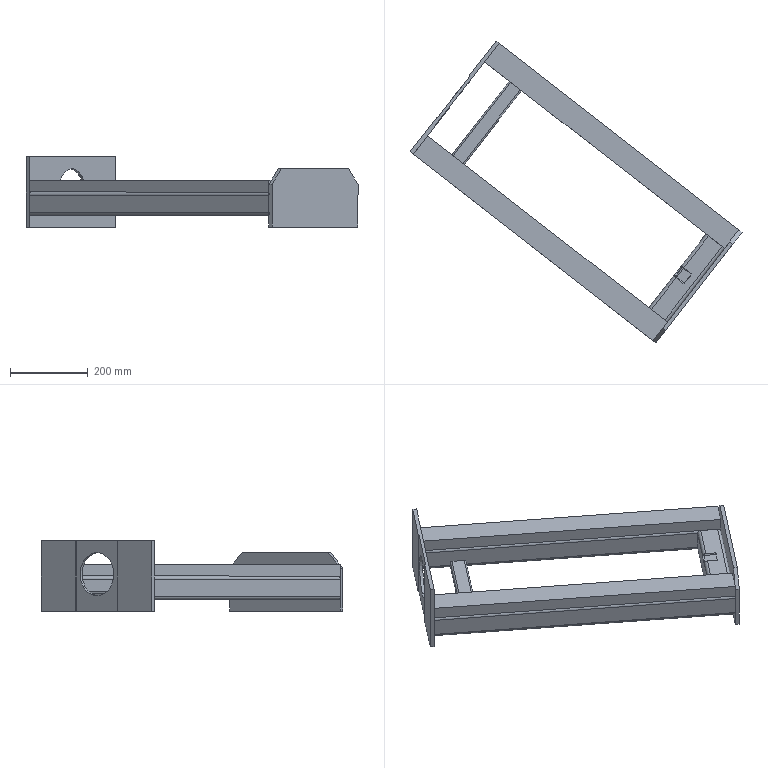Component | SolidWorks | MotorMountingPlate-1 | 8 solids | 109 faces | box 852.7 x 774.93 x 180 mm | volume 5440747 mm3 | plane 71 | cylinder 38 | commonest cylinder face diameters 8 x17 16 x13 4 x4 34 x2 110.02 x2
build123d program:
from build123d import *

# Parameters (mm, degrees)
SQUARE_TUBE_60_X_60_X_4_0_1_DEPTH      = 750
SQUARE_TUBE_60_X_60_X_4_0_1_DEPTH_BACK = 30
SQUARE_TUBE_60_X_60_X_4_0_1_2_DEPTH    = 780
SQUARE_TUBE_60_X_60_X_4_0_1_3_DEPTH    = 302
SKETCH2_W                              = 360
SKETCH2_H                              = 180
BOSS_EXTRUDE1_DEPTH                    = 10
SKETCH3_W                              = 360
SKETCH3_H                              = 150
BOSS_EXTRUDE2_DEPTH                    = 10
CHAMFER1_SIZE                          = 40
SKETCH4_W                              = 135
SKETCH4_H                              = 180
CUT_EXTRUDE2_2_DEPTH                   = 2
SKETCH6_R                              = 55.01
CUT_EXTRUDE3_2_DEPTH                   = 8
SKETCH7_W                              = 60
SKETCH7_H                              = 780
BOSS_EXTRUDE3_DEPTH                    = 30
BOSS_EXTRUDE3_2_DEPTH                  = 30
RECTANGULAR_TUBE_40X20X2_1_DEPTH       = 300
CUT_EXTRUDE2_DEPTH                     = 31
CUT_EXTRUDE2_DEPTH_BACK                = 4
SKETCH13_R                             = 17
CUT_EXTRUDE3_DEPTH                     = 35
CUT_EXTRUDE3_DEPTH_BACK                = 35
SKETCH12_W                             = 65
SKETCH12_H                             = 50


with BuildPart() as part:
    # Sketch11 → Square Tube 60 X 60 X 4.0-_1 (new, two sides: drawn at the far end of the back side and taken through both)
    with BuildSketch(Plane(origin=(0, 0, 0), x_dir=(1, 0, 0), z_dir=(0, 1, 0)).offset(-SQUARE_TUBE_60_X_60_X_4_0_1_DEPTH_BACK)):
        with BuildLine():
            Line((-22, -30), (22, -30))
            ThreePointArc((22, -30), (27.657, -27.657), (30, -22))
            Line((30, -22), (30, 22))
            ThreePointArc((30, 22), (27.657, 27.657), (22, 30))
            Line((22, 30), (-22, 30))
            ThreePointArc((-22, 30), (-27.657, 27.657), (-30, 22))
            Line((-30, 22), (-30, -22))
            ThreePointArc((-30, -22), (-27.657, -27.657), (-22, -30))
        make_face()
        with BuildLine():
            Line((-22, -26), (22, -26))
            ThreePointArc((22, -26), (24.828, -24.828), (26, -22))
            Line((26, -22), (26, 22))
            ThreePointArc((26, 22), (24.828, 24.828), (22, 26))
            Line((22, 26), (-22, 26))
            ThreePointArc((-22, 26), (-24.828, 24.828), (-26, 22))
            Line((-26, 22), (-26, -22))
            ThreePointArc((-26, -22), (-24.828, -24.828), (-22, -26))
        make_face(mode=Mode.SUBTRACT)
    extrude(amount=SQUARE_TUBE_60_X_60_X_4_0_1_DEPTH + SQUARE_TUBE_60_X_60_X_4_0_1_DEPTH_BACK)


with BuildPart() as body_2:
    # Sketch11 on segment 2 (on carried to segment 2) → Square Tube 60 X 60 X 4.0-_1 2 (new body)
    with BuildSketch(Plane(origin=(300, -30, 0), x_dir=(1, 0, 0), z_dir=(0, 1, 0))):
        with BuildLine():
            Line((-22, -30), (22, -30))
            ThreePointArc((22, -30), (27.657, -27.657), (30, -22))
            Line((30, -22), (30, 22))
            ThreePointArc((30, 22), (27.657, 27.657), (22, 30))
            Line((22, 30), (-22, 30))
            ThreePointArc((-22, 30), (-27.657, 27.657), (-30, 22))
            Line((-30, 22), (-30, -22))
            ThreePointArc((-30, -22), (-27.657, -27.657), (-22, -30))
        make_face()
        with BuildLine():
            Line((-22, -26), (22, -26))
            ThreePointArc((22, -26), (24.828, -24.828), (26, -22))
            Line((26, -22), (26, 22))
            ThreePointArc((26, 22), (24.828, 24.828), (22, 26))
            Line((22, 26), (-22, 26))
            ThreePointArc((-22, 26), (-24.828, 24.828), (-26, 22))
            Line((-26, 22), (-26, -22))
            ThreePointArc((-26, -22), (-24.828, -24.828), (-22, -26))
        make_face(mode=Mode.SUBTRACT)
    extrude(amount=SQUARE_TUBE_60_X_60_X_4_0_1_2_DEPTH)


with BuildPart() as body_3:
    # Sketch11 on segment 3 (on carried to segment 3) → Square Tube 60 X 60 X 4.0-_1 3 (new body)
    with BuildSketch(Plane(origin=(-1, 0, 0), x_dir=(0, -1, 0), z_dir=(1, 0, 0))):
        with BuildLine():
            Line((-22, -30), (22, -30))
            ThreePointArc((22, -30), (27.657, -27.657), (30, -22))
            Line((30, -22), (30, 22))
            ThreePointArc((30, 22), (27.657, 27.657), (22, 30))
            Line((22, 30), (-22, 30))
            ThreePointArc((-22, 30), (-27.657, 27.657), (-30, 22))
            Line((-30, 22), (-30, -22))
            ThreePointArc((-30, -22), (-27.657, -27.657), (-22, -30))
        make_face()
        with BuildLine():
            Line((-22, -26), (22, -26))
            ThreePointArc((22, -26), (24.828, -24.828), (26, -22))
            Line((26, -22), (26, 22))
            ThreePointArc((26, 22), (24.828, 24.828), (22, 26))
            Line((22, 26), (-22, 26))
            ThreePointArc((-22, 26), (-24.828, 24.828), (-26, 22))
            Line((-26, 22), (-26, -22))
            ThreePointArc((-26, -22), (-24.828, -24.828), (-22, -26))
        make_face(mode=Mode.SUBTRACT)
    extrude(amount=SQUARE_TUBE_60_X_60_X_4_0_1_3_DEPTH)

    # Square Tube 60 X 60 X 4.0-_1 3 end butt
    split(bisect_by=Plane.YZ.offset(30), keep=Keep.TOP)

    # Square Tube 60 X 60 X 4.0-_1 3 end b 2
    split(bisect_by=Plane(origin=(270, 0, 0), x_dir=(0, -1, 0), z_dir=(-1, 0, 0)), keep=Keep.TOP)

    # Sketch13 → Cut-Extrude2 (cut, two sides: drawn at the far end of the back side and taken through both)
    with BuildSketch(Plane(origin=(0, 0, 0), x_dir=(1, 0, 0), z_dir=(0, 1, 0)).offset(-CUT_EXTRUDE2_DEPTH_BACK)):
        with Locations((150, 35)):
            Circle(SKETCH13_R)
    extrude(amount=CUT_EXTRUDE2_DEPTH + CUT_EXTRUDE2_DEPTH_BACK, mode=Mode.SUBTRACT)


with BuildPart() as body_4:
    # Sketch2 → Boss-Extrude1 (new body)
    with BuildSketch(Plane(origin=(0, 750, 0), x_dir=(1, 0, 0), z_dir=(0, 1, 0))):
        with Locations((150, 30)):
            Rectangle(SKETCH2_W, SKETCH2_H)
    extrude(amount=BOSS_EXTRUDE1_DEPTH)

    # Sketch4 → Cut-Extrude2_2 (cut)
    with BuildSketch(Plane(origin=(0, 760, 0), x_dir=(1, 0, 0), z_dir=(0, 1, 0))):
        with Locations((150, 30)):
            Rectangle(SKETCH4_W, SKETCH4_H)
    extrude(amount=-CUT_EXTRUDE2_2_DEPTH, mode=Mode.SUBTRACT)

    # Sketch6 → Cut-Extrude3_2 (cut)
    with BuildSketch(Plane(origin=(0, 758, 0), x_dir=(1, 0, 0), z_dir=(0, 1, 0))):
        with Locations(Location((150, 35, 0), (0, 0, 270))):
            Circle(SKETCH6_R)
    extrude(amount=-CUT_EXTRUDE3_2_DEPTH, mode=Mode.SUBTRACT)


with BuildPart() as body_5:
    # Sketch3 → Boss-Extrude2 (new body)
    with BuildSketch(Plane.XZ.offset(30)):
        with Locations((150, -15)):
            Rectangle(SKETCH3_W, SKETCH3_H)
    extrude(amount=BOSS_EXTRUDE2_DEPTH)

    # Chamfer1
    chamfer1_edges = [body_5.edges().sort_by_distance(p)[0] for p in [
        (330, -35, -90),
        (-30, -35, -90),
    ]]
    chamfer(chamfer1_edges, length=CHAMFER1_SIZE)


with BuildPart() as body_6:
    # Sketch7 → Boss-Extrude3 (new body)
    with BuildSketch(Plane(origin=(0, 0, -30), x_dir=(-1, 0, 0), z_dir=(0, 0, -1))):
        with Locations((0, 360)):
            Rectangle(SKETCH7_W, SKETCH7_H)
    extrude(amount=BOSS_EXTRUDE3_DEPTH)


with BuildPart() as body_7:
    # Sketch7 → Boss-Extrude3 2 (new body)
    with BuildSketch(Plane(origin=(0, 0, -30), x_dir=(-1, 0, 0), z_dir=(0, 0, -1))):
        with Locations((-300, 360)):
            Rectangle(SKETCH7_W, SKETCH7_H)
    extrude(amount=BOSS_EXTRUDE3_2_DEPTH)


with BuildPart() as body_8:
    # Sketch1 → Rectangular Tube 40X20X2-_1 (new body)
    with BuildSketch(Plane(origin=(0, 650, 20), x_dir=(0, 0, -1), z_dir=(1, 0, 0))):
        with BuildLine():
            Line((-6, -20), (6, -20))
            ThreePointArc((6, -20), (8.828, -18.828), (10, -16))
            Line((10, -16), (10, 16))
            ThreePointArc((10, 16), (8.828, 18.828), (6, 20))
            Line((6, 20), (-6, 20))
            ThreePointArc((-6, 20), (-8.828, 18.828), (-10, 16))
            Line((-10, 16), (-10, -16))
            ThreePointArc((-10, -16), (-8.828, -18.828), (-6, -20))
        make_face()
        with BuildLine():
            Line((-6, -18), (6, -18))
            ThreePointArc((6, -18), (7.414, -17.414), (8, -16))
            Line((8, -16), (8, 16))
            ThreePointArc((8, 16), (7.414, 17.414), (6, 18))
            Line((6, 18), (-6, 18))
            ThreePointArc((-6, 18), (-7.414, 17.414), (-8, 16))
            Line((-8, 16), (-8, -16))
            ThreePointArc((-8, -16), (-7.414, -17.414), (-6, -18))
        make_face(mode=Mode.SUBTRACT)
    extrude(amount=RECTANGULAR_TUBE_40X20X2_1_DEPTH)

    # Sketch12 → Cut-Extrude3 (cut, two sides: drawn at the far end of the back side and taken through both)
    with BuildSketch(Plane.XY.offset(-CUT_EXTRUDE3_DEPTH_BACK)):
        with Locations((-2.5, 650)):
            Rectangle(SKETCH12_W, SKETCH12_H)
        with Locations((302.5, 650)):
            Rectangle(SKETCH12_W, SKETCH12_H)
    extrude(amount=CUT_EXTRUDE3_DEPTH + CUT_EXTRUDE3_DEPTH_BACK, mode=Mode.SUBTRACT)


solid = Compound([part.part, body_2.part, body_3.part, body_4.part, body_5.part, body_6.part, body_7.part, body_8.part])

# Placed as in the assembly
solid = solid.moved(Location((472.655, 567.626, 241.411), (-180, 0, 127.821)))